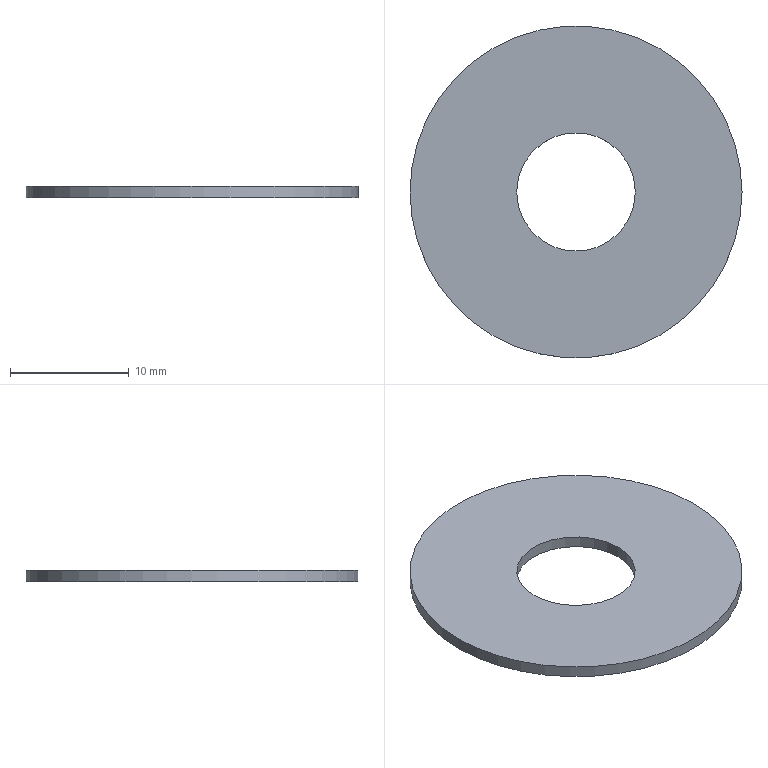Component | NX | WASHER | 1 solid | 4 faces | box 28 x 28 x 1 mm | volume 537 mm3 | cylinder 2 | plane 2 | commonest cylinder face diameters 28 x1 10 x1
STEP:
#1=CARTESIAN_POINT('',(0.,0.,0.));
#2=DIRECTION('',(0.,0.,1.));
#3=DIRECTION('',(1.,0.,0.));
#4=AXIS2_PLACEMENT_3D('',#1,#2,#3);
#5=CARTESIAN_POINT('',(103.996,70.391,11.));
#6=VERTEX_POINT('',#5);
#7=CARTESIAN_POINT('',(89.996,70.391,11.));
#8=DIRECTION('',(0.,0.,1.));
#9=DIRECTION('',(1.,0.,0.));
#10=AXIS2_PLACEMENT_3D('',#7,#8,#9);
#11=CIRCLE('',#10,14.);
#12=CARTESIAN_POINT('',(89.996,70.391,11.));
#13=DIRECTION('',(0.,0.,-1.));
#14=DIRECTION('',(-1.,0.,0.));
#15=AXIS2_PLACEMENT_3D('',#12,#13,#14);
#16=CYLINDRICAL_SURFACE('',#15,14.);
#17=CARTESIAN_POINT('',(9.425,0.));
#18=DIRECTION('',(-1.,0.));
#19=VECTOR('',#18,1.);
#20=LINE('',#17,#19);
#21=(GEOMETRIC_REPRESENTATION_CONTEXT(2)PARAMETRIC_REPRESENTATION_CONTEXT()REPRESENTATION_CONTEXT('',''));
#22=DEFINITIONAL_REPRESENTATION('',(#20),#21);
#23=PCURVE('',#16,#22);
#24=CARTESIAN_POINT('',(89.996,70.391,11.));
#25=DIRECTION('',(0.,0.,1.));
#26=DIRECTION('',(1.,0.,0.));
#27=AXIS2_PLACEMENT_3D('',#24,#25,#26);
#28=PLANE('',#27);
#29=CARTESIAN_POINT('',(0.,0.));
#30=DIRECTION('',(1.,0.));
#31=AXIS2_PLACEMENT_2D('',#29,#30);
#32=CIRCLE('',#31,14.);
#33=(GEOMETRIC_REPRESENTATION_CONTEXT(2)PARAMETRIC_REPRESENTATION_CONTEXT()REPRESENTATION_CONTEXT('',''));
#34=DEFINITIONAL_REPRESENTATION('',(#32),#33);
#35=PCURVE('',#28,#34);
#36=SURFACE_CURVE('',#11,(#23,#35),.PCURVE_S1.);
#37=EDGE_CURVE('',#6,#6,#36,.T.);
#38=ORIENTED_EDGE('',*,*,#37,.F.);
#39=CARTESIAN_POINT('',(103.996,70.391,10.));
#40=VERTEX_POINT('',#39);
#41=CARTESIAN_POINT('',(103.996,70.391,11.));
#42=CARTESIAN_POINT('',(103.996,70.391,10.));
#43=B_SPLINE_CURVE_WITH_KNOTS('',1,(#41,#42),.UNSPECIFIED.,.F.,.F.,(2,2),(0.,1.),.PIECEWISE_BEZIER_KNOTS.);
#44=CARTESIAN_POINT('',(9.425,0.));
#45=DIRECTION('',(0.,1.));
#46=VECTOR('',#45,1.);
#47=LINE('',#44,#46);
#48=(GEOMETRIC_REPRESENTATION_CONTEXT(2)PARAMETRIC_REPRESENTATION_CONTEXT()REPRESENTATION_CONTEXT('',''));
#49=DEFINITIONAL_REPRESENTATION('',(#47),#48);
#50=PCURVE('',#16,#49);
#51=CARTESIAN_POINT('',(3.142,0.));
#52=DIRECTION('',(0.,1.));
#53=VECTOR('',#52,1.);
#54=LINE('',#51,#53);
#55=(GEOMETRIC_REPRESENTATION_CONTEXT(2)PARAMETRIC_REPRESENTATION_CONTEXT()REPRESENTATION_CONTEXT('',''));
#56=DEFINITIONAL_REPRESENTATION('',(#54),#55);
#57=PCURVE('',#16,#56);
#58=SEAM_CURVE('',#43,(#50,#57),.PCURVE_S1.);
#59=EDGE_CURVE('',#6,#40,#58,.T.);
#60=ORIENTED_EDGE('',*,*,#59,.T.);
#61=CARTESIAN_POINT('',(89.996,70.391,10.));
#62=DIRECTION('',(0.,0.,1.));
#63=DIRECTION('',(1.,0.,0.));
#64=AXIS2_PLACEMENT_3D('',#61,#62,#63);
#65=CIRCLE('',#64,14.);
#66=CARTESIAN_POINT('',(9.425,1.));
#67=DIRECTION('',(-1.,0.));
#68=VECTOR('',#67,1.);
#69=LINE('',#66,#68);
#70=(GEOMETRIC_REPRESENTATION_CONTEXT(2)PARAMETRIC_REPRESENTATION_CONTEXT()REPRESENTATION_CONTEXT('',''));
#71=DEFINITIONAL_REPRESENTATION('',(#69),#70);
#72=PCURVE('',#16,#71);
#73=CARTESIAN_POINT('',(89.996,70.391,10.));
#74=DIRECTION('',(0.,0.,1.));
#75=DIRECTION('',(1.,0.,0.));
#76=AXIS2_PLACEMENT_3D('',#73,#74,#75);
#77=PLANE('',#76);
#78=CARTESIAN_POINT('',(0.,0.));
#79=DIRECTION('',(1.,0.));
#80=AXIS2_PLACEMENT_2D('',#78,#79);
#81=CIRCLE('',#80,14.);
#82=(GEOMETRIC_REPRESENTATION_CONTEXT(2)PARAMETRIC_REPRESENTATION_CONTEXT()REPRESENTATION_CONTEXT('',''));
#83=DEFINITIONAL_REPRESENTATION('',(#81),#82);
#84=PCURVE('',#77,#83);
#85=SURFACE_CURVE('',#65,(#72,#84),.PCURVE_S1.);
#86=EDGE_CURVE('',#40,#40,#85,.T.);
#87=ORIENTED_EDGE('',*,*,#86,.T.);
#88=ORIENTED_EDGE('',*,*,#59,.F.);
#89=EDGE_LOOP('',(#38,#60,#87,#88));
#90=FACE_BOUND('',#89,.T.);
#91=ADVANCED_FACE('',(#90),#16,.T.);
#92=CARTESIAN_POINT('',(94.996,70.391,11.));
#93=VERTEX_POINT('',#92);
#94=CARTESIAN_POINT('',(89.996,70.391,11.));
#95=DIRECTION('',(0.,0.,-1.));
#96=DIRECTION('',(1.,0.,0.));
#97=AXIS2_PLACEMENT_3D('',#94,#95,#96);
#98=CIRCLE('',#97,5.);
#99=CARTESIAN_POINT('',(89.996,70.391,11.));
#100=DIRECTION('',(0.,0.,-1.));
#101=DIRECTION('',(-1.,0.,0.));
#102=AXIS2_PLACEMENT_3D('',#99,#100,#101);
#103=CYLINDRICAL_SURFACE('',#102,5.);
#104=CARTESIAN_POINT('',(3.142,0.));
#105=DIRECTION('',(1.,0.));
#106=VECTOR('',#105,1.);
#107=LINE('',#104,#106);
#108=(GEOMETRIC_REPRESENTATION_CONTEXT(2)PARAMETRIC_REPRESENTATION_CONTEXT()REPRESENTATION_CONTEXT('',''));
#109=DEFINITIONAL_REPRESENTATION('',(#107),#108);
#110=PCURVE('',#103,#109);
#111=CARTESIAN_POINT('',(5.,0.));
#112=CARTESIAN_POINT('',(5.,-8.66));
#113=CARTESIAN_POINT('',(-2.5,-4.33));
#114=CARTESIAN_POINT('',(-10.,-0.));
#115=CARTESIAN_POINT('',(-2.5,4.33));
#116=CARTESIAN_POINT('',(5.,8.66));
#117=CARTESIAN_POINT('',(5.,0.));
#118=(BOUNDED_CURVE()B_SPLINE_CURVE(2,(#111,#112,#113,#114,#115,#116,#117),.UNSPECIFIED.,.T.,.F.)B_SPLINE_CURVE_WITH_KNOTS((1,2,2,2,2,1),(-2.094,0.,2.094,4.189,6.283,8.378),.UNSPECIFIED.)CURVE()GEOMETRIC_REPRESENTATION_ITEM()RATIONAL_B_SPLINE_CURVE((1.,0.5,1.,0.5,1.,0.5,1.))REPRESENTATION_ITEM(''));
#119=(GEOMETRIC_REPRESENTATION_CONTEXT(2)PARAMETRIC_REPRESENTATION_CONTEXT()REPRESENTATION_CONTEXT('',''));
#120=DEFINITIONAL_REPRESENTATION('',(#118),#119);
#121=PCURVE('',#28,#120);
#122=SURFACE_CURVE('',#98,(#110,#121),.PCURVE_S1.);
#123=EDGE_CURVE('',#93,#93,#122,.T.);
#124=ORIENTED_EDGE('',*,*,#123,.T.);
#125=CARTESIAN_POINT('',(94.996,70.391,10.));
#126=VERTEX_POINT('',#125);
#127=CARTESIAN_POINT('',(94.996,70.391,11.));
#128=CARTESIAN_POINT('',(94.996,70.391,10.));
#129=B_SPLINE_CURVE_WITH_KNOTS('',1,(#127,#128),.UNSPECIFIED.,.F.,.F.,(2,2),(0.,1.),.PIECEWISE_BEZIER_KNOTS.);
#130=CARTESIAN_POINT('',(9.425,0.));
#131=DIRECTION('',(0.,1.));
#132=VECTOR('',#131,1.);
#133=LINE('',#130,#132);
#134=(GEOMETRIC_REPRESENTATION_CONTEXT(2)PARAMETRIC_REPRESENTATION_CONTEXT()REPRESENTATION_CONTEXT('',''));
#135=DEFINITIONAL_REPRESENTATION('',(#133),#134);
#136=PCURVE('',#103,#135);
#137=CARTESIAN_POINT('',(3.142,0.));
#138=DIRECTION('',(0.,1.));
#139=VECTOR('',#138,1.);
#140=LINE('',#137,#139);
#141=(GEOMETRIC_REPRESENTATION_CONTEXT(2)PARAMETRIC_REPRESENTATION_CONTEXT()REPRESENTATION_CONTEXT('',''));
#142=DEFINITIONAL_REPRESENTATION('',(#140),#141);
#143=PCURVE('',#103,#142);
#144=SEAM_CURVE('',#129,(#136,#143),.PCURVE_S1.);
#145=EDGE_CURVE('',#93,#126,#144,.T.);
#146=ORIENTED_EDGE('',*,*,#145,.T.);
#147=CARTESIAN_POINT('',(89.996,70.391,10.));
#148=DIRECTION('',(0.,0.,-1.));
#149=DIRECTION('',(1.,0.,0.));
#150=AXIS2_PLACEMENT_3D('',#147,#148,#149);
#151=CIRCLE('',#150,5.);
#152=CARTESIAN_POINT('',(3.142,1.));
#153=DIRECTION('',(1.,0.));
#154=VECTOR('',#153,1.);
#155=LINE('',#152,#154);
#156=(GEOMETRIC_REPRESENTATION_CONTEXT(2)PARAMETRIC_REPRESENTATION_CONTEXT()REPRESENTATION_CONTEXT('',''));
#157=DEFINITIONAL_REPRESENTATION('',(#155),#156);
#158=PCURVE('',#103,#157);
#159=CARTESIAN_POINT('',(5.,0.));
#160=CARTESIAN_POINT('',(5.,-8.66));
#161=CARTESIAN_POINT('',(-2.5,-4.33));
#162=CARTESIAN_POINT('',(-10.,-0.));
#163=CARTESIAN_POINT('',(-2.5,4.33));
#164=CARTESIAN_POINT('',(5.,8.66));
#165=CARTESIAN_POINT('',(5.,0.));
#166=(BOUNDED_CURVE()B_SPLINE_CURVE(2,(#159,#160,#161,#162,#163,#164,#165),.UNSPECIFIED.,.T.,.F.)B_SPLINE_CURVE_WITH_KNOTS((1,2,2,2,2,1),(-2.094,0.,2.094,4.189,6.283,8.378),.UNSPECIFIED.)CURVE()GEOMETRIC_REPRESENTATION_ITEM()RATIONAL_B_SPLINE_CURVE((1.,0.5,1.,0.5,1.,0.5,1.))REPRESENTATION_ITEM(''));
#167=(GEOMETRIC_REPRESENTATION_CONTEXT(2)PARAMETRIC_REPRESENTATION_CONTEXT()REPRESENTATION_CONTEXT('',''));
#168=DEFINITIONAL_REPRESENTATION('',(#166),#167);
#169=PCURVE('',#77,#168);
#170=SURFACE_CURVE('',#151,(#158,#169),.PCURVE_S1.);
#171=EDGE_CURVE('',#126,#126,#170,.T.);
#172=ORIENTED_EDGE('',*,*,#171,.F.);
#173=ORIENTED_EDGE('',*,*,#145,.F.);
#174=EDGE_LOOP('',(#124,#146,#172,#173));
#175=FACE_BOUND('',#174,.F.);
#176=ADVANCED_FACE('',(#175),#103,.F.);
#177=ORIENTED_EDGE('',*,*,#37,.T.);
#178=EDGE_LOOP('',(#177));
#179=FACE_BOUND('',#178,.T.);
#180=ORIENTED_EDGE('',*,*,#123,.T.);
#181=EDGE_LOOP('',(#180));
#182=FACE_BOUND('',#181,.T.);
#183=ADVANCED_FACE('',(#179,#182),#28,.T.);
#184=ORIENTED_EDGE('',*,*,#86,.F.);
#185=EDGE_LOOP('',(#184));
#186=FACE_BOUND('',#185,.T.);
#187=ORIENTED_EDGE('',*,*,#171,.F.);
#188=EDGE_LOOP('',(#187));
#189=FACE_BOUND('',#188,.T.);
#190=ADVANCED_FACE('',(#186,#189),#77,.F.);
#191=CLOSED_SHELL('',(#91,#176,#183,#190));
#192=MANIFOLD_SOLID_BREP('',#191);
#193=(LENGTH_UNIT()NAMED_UNIT(*)SI_UNIT(.MILLI.,.METRE.));
#194=UNCERTAINTY_MEASURE_WITH_UNIT(LENGTH_MEASURE(0.00001),#193,'','');
#195=(NAMED_UNIT(*)PLANE_ANGLE_UNIT()SI_UNIT($,.RADIAN.));
#196=(NAMED_UNIT(*)SI_UNIT($,.STERADIAN.)SOLID_ANGLE_UNIT());
#197=(GEOMETRIC_REPRESENTATION_CONTEXT(3)GLOBAL_UNCERTAINTY_ASSIGNED_CONTEXT((#194))GLOBAL_UNIT_ASSIGNED_CONTEXT((#193,#195,#196))REPRESENTATION_CONTEXT('',''));
#198=ADVANCED_BREP_SHAPE_REPRESENTATION('',(#4,#192),#197);